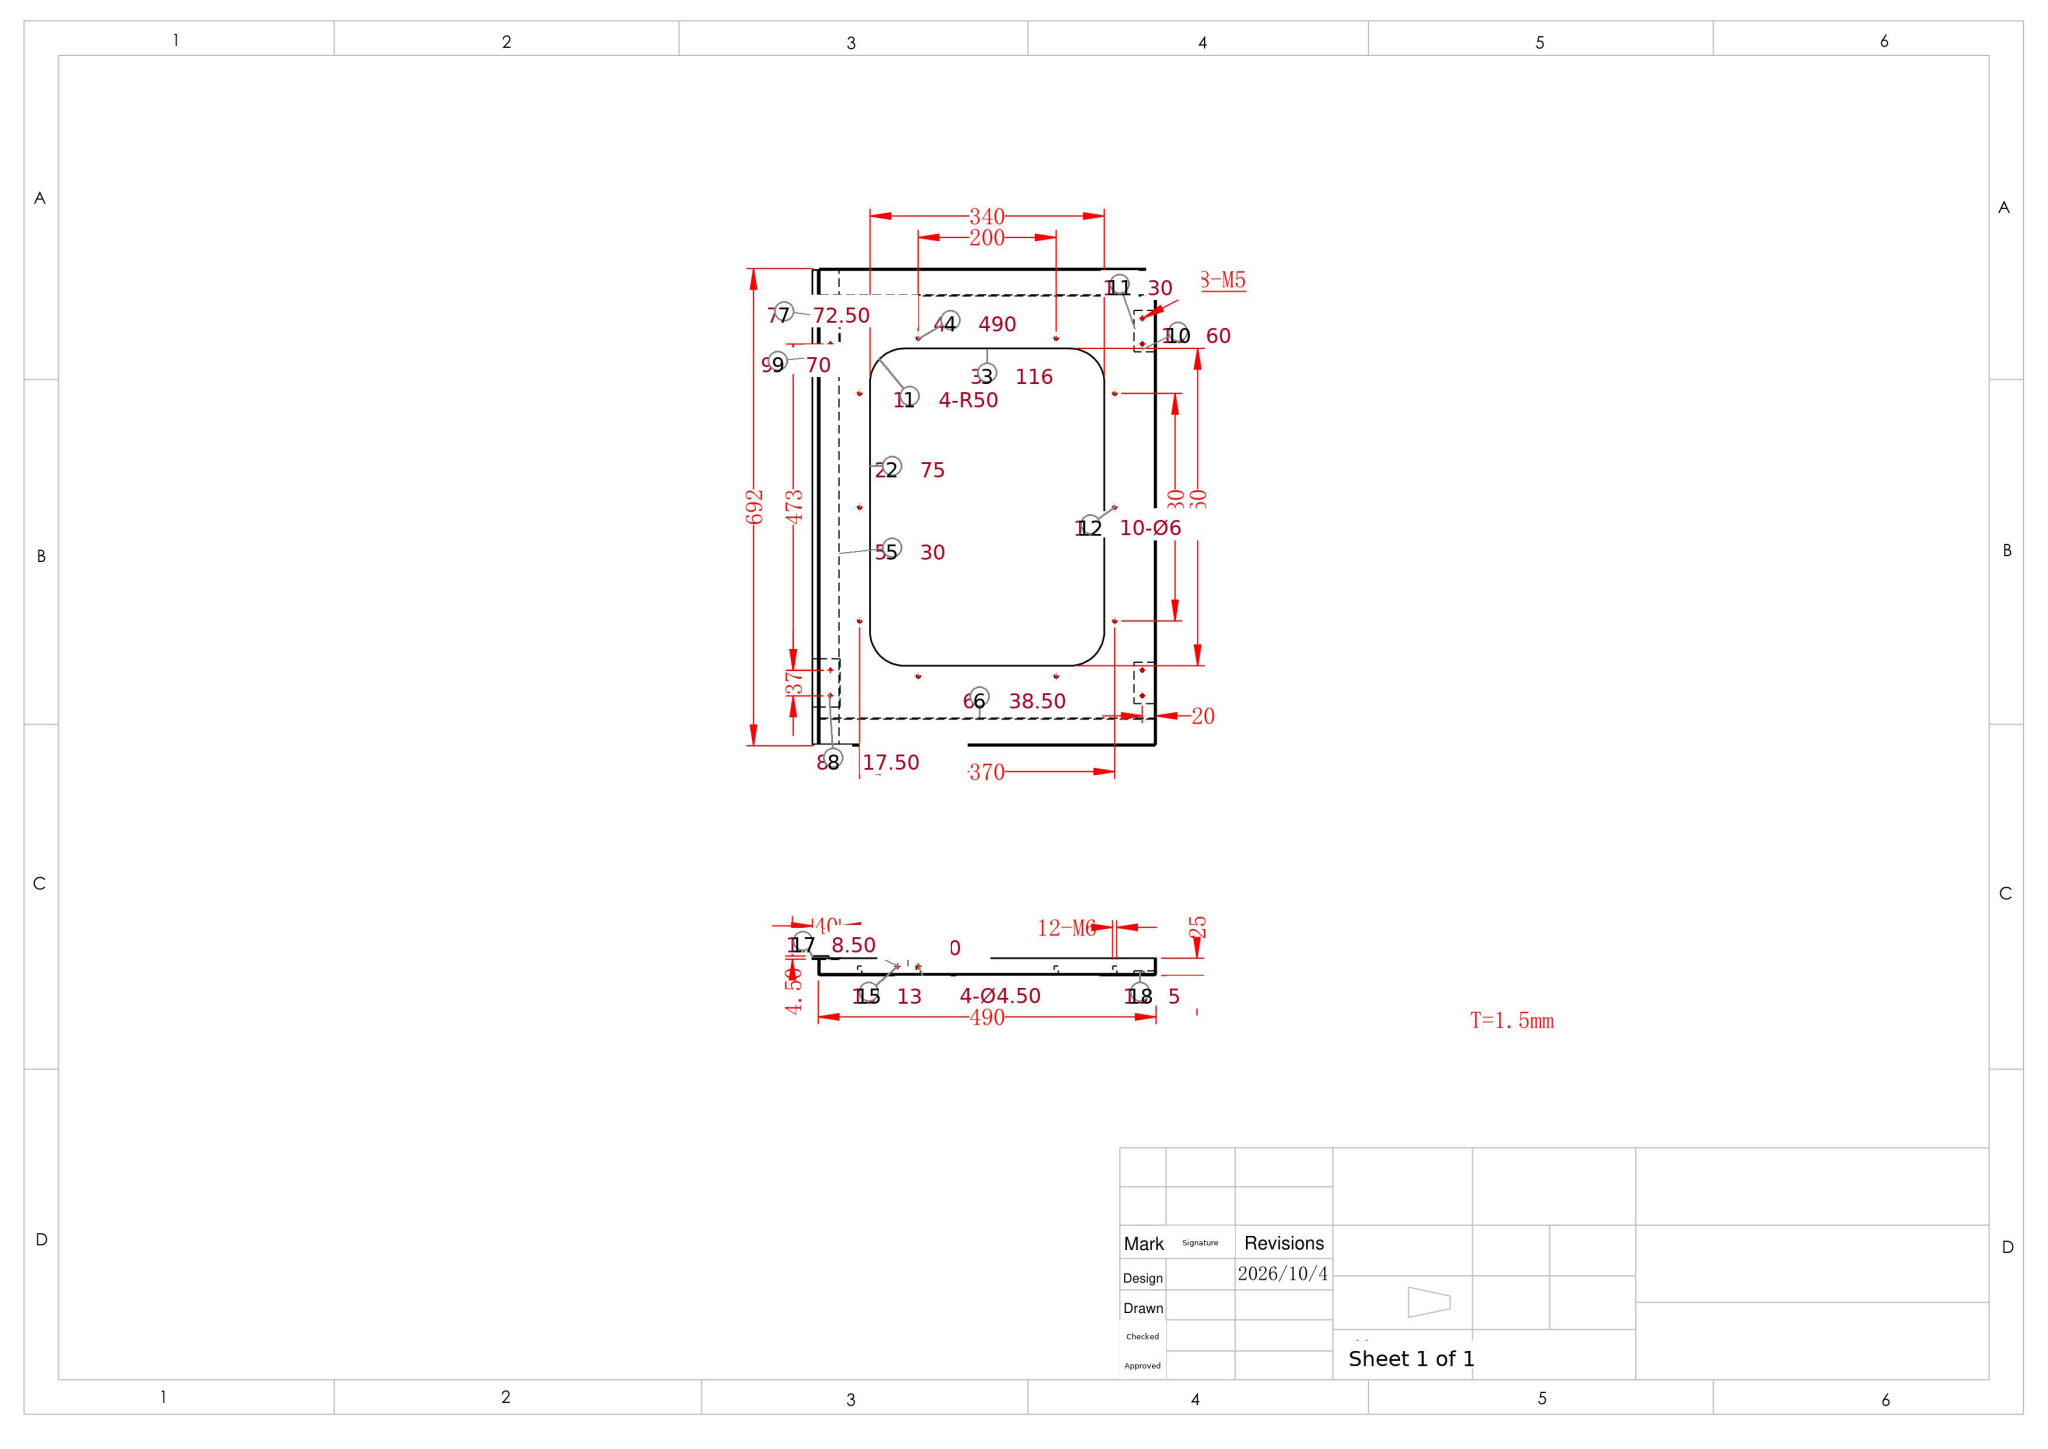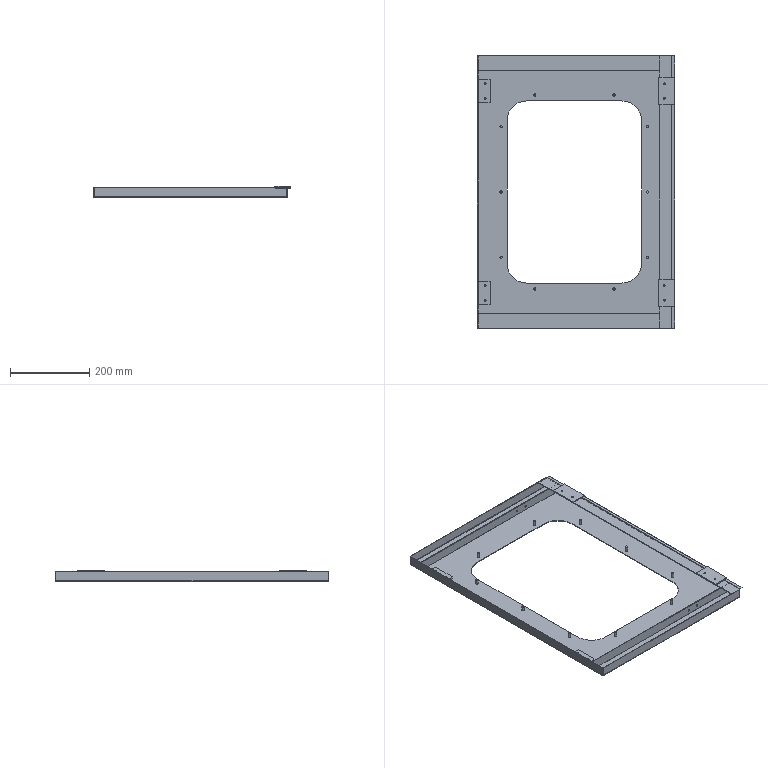Part | SolidWorks | mm | 1 solid | 151 faces | box 498.5 x 692 x 28 mm | volume 477256 mm3 | plane 84 | cylinder 59 | spline 8 | commonest cylinder face diameters 6 x20 4.2 x16 4.5 x8 4.473 x6 1.473 x5 100 x4